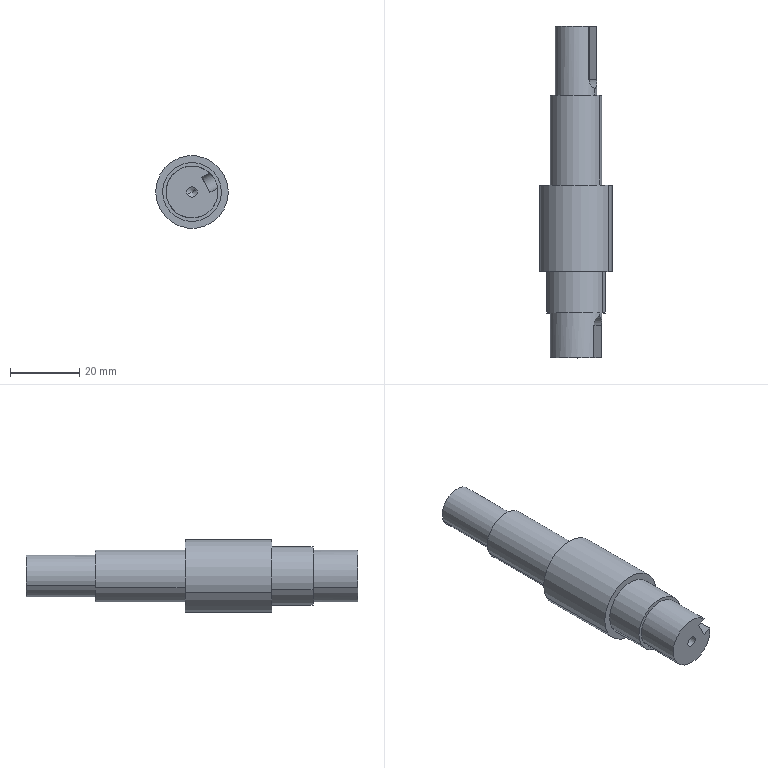Component | SolidWorks | GearIntermediateAxis-1 | 1 solid | 32 faces | box 21 x 96 x 21 mm | volume 19909 mm3 | cylinder 16 | plane 12 | cone 4 | commonest cylinder face diameters 3 x4 15 x4 17 x2 21 x2 12 x2 5 x2 | material 5154-O, Bar (SS)
build123d program:
from build123d import *

# Parameters (mm, degrees)
CUT_EXTRUDE1_DEPTH    = 3
CUT_EXTRUDE2_DEPTH    = 3
M3_TAPPED_HOLE1_D     = 3
M3_TAPPED_HOLE1_DEPTH = 15
M3_TAPPED_HOLE1_TIP   = 0.9013
M3_TAPPED_HOLE2_D     = 3
M3_TAPPED_HOLE2_DEPTH = 15
M3_TAPPED_HOLE2_TIP   = 0.9013


with BuildPart() as part:
    # Sketch1 → Revolve1 (revolve)
    with BuildSketch(Plane.XY, mode=Mode.PRIVATE) as revolve1_sk:
        Polygon((0, 96), (-6, 96), (-6, 76), (-7.5, 76), (-7.5, 50), (-10.5, 50), (-10.5, 25), (-8.5, 25), (-8.5, 13), (-7.5, 13), (-7.5, 0), (0, 0), align=None)
    revolve(revolve1_sk.sketch.rotate(Axis((0, 111.479, 0), (0, -1, 0)), 270), axis=Axis((0, 111.479, 0), (0, -1, 0)))

    # Sketch2 → Cut-Extrude1 (cut)
    with BuildSketch(Plane.XY.offset(6)):
        with BuildLine():
            Line((2.5, 96), (2.5, 80.5))
            ThreePointArc((2.5, 80.5), (0, 78), (-2.5, 80.5))
            Line((-2.5, 80.5), (-2.5, 96))
            ThreePointArc((-2.5, 96), (0, 98.5), (2.5, 96))
        make_face()
    extrude(amount=-CUT_EXTRUDE1_DEPTH, mode=Mode.SUBTRACT)

    # Sketch3 → Cut-Extrude2 (cut)
    with BuildSketch(Plane.XY.offset(7.5)):
        with BuildLine():
            Line((-2.5, 0), (-2.5, 9.5))
            ThreePointArc((-2.5, 9.5), (0, 12), (2.5, 9.5))
            Line((2.5, 9.5), (2.5, 0))
            ThreePointArc((2.5, 0), (0, -2.5), (-2.5, 0))
        make_face()
    extrude(amount=-CUT_EXTRUDE2_DEPTH, mode=Mode.SUBTRACT)

    # M3 Tapped Hole1
    with Locations(Plane(origin=(0, 96, 0), x_dir=(1, 0, 0), z_dir=(0, 1, 0))):
        with Locations((0, 0)):
            Hole(M3_TAPPED_HOLE1_D / 2, depth=M3_TAPPED_HOLE1_DEPTH)
            with Locations((0, 0, -(M3_TAPPED_HOLE1_DEPTH + M3_TAPPED_HOLE1_TIP / 2))):  # 118° drill point
                Cone(0, M3_TAPPED_HOLE1_D / 2, M3_TAPPED_HOLE1_TIP, mode=Mode.SUBTRACT)

    # M3 Tapped Hole2
    with Locations(Plane(origin=(0, 0, 0), x_dir=(-1, 0, 0), z_dir=(0, -1, 0))):
        with Locations((0, 0)):
            Hole(M3_TAPPED_HOLE2_D / 2, depth=M3_TAPPED_HOLE2_DEPTH)
            with Locations((0, 0, -(M3_TAPPED_HOLE2_DEPTH + M3_TAPPED_HOLE2_TIP / 2))):  # 118° drill point
                Cone(0, M3_TAPPED_HOLE2_D / 2, M3_TAPPED_HOLE2_TIP, mode=Mode.SUBTRACT)


solid = part.part

# Placed as in the assembly
solid = solid.moved(Location((-165.724, 61.266, -166.507), (0, 62.569, 0)))
STEP:
#1=COLOUR_RGB('',0.7922,0.8196,0.9333);
#2=FILL_AREA_STYLE_COLOUR('',#1);
#3=FILL_AREA_STYLE('',(#2));
#4=SURFACE_STYLE_FILL_AREA(#3);
#5=SURFACE_SIDE_STYLE('',(#4));
#6=SURFACE_STYLE_USAGE(.BOTH.,#5);
#7=PRESENTATION_STYLE_ASSIGNMENT((#6));
#8=CARTESIAN_POINT('',(-6.472,3.003,-6.528));
#9=VERTEX_POINT('',#8);
#10=CARTESIAN_POINT('',(-6.577,3.003,-6.583));
#11=VERTEX_POINT('',#10);
#12=CARTESIAN_POINT('',(-6.525,3.003,-6.555));
#13=DIRECTION('',(0.,-1.,0.));
#14=DIRECTION('',(-0.8876,0.,-0.4607));
#15=AXIS2_PLACEMENT_3D('',#12,#13,#14);
#16=CIRCLE('',#15,0.05906);
#17=EDGE_CURVE('',#9,#11,#16,.T.);
#18=ORIENTED_EDGE('',*,*,#17,.F.);
#19=CARTESIAN_POINT('',(-6.472,2.412,-6.528));
#20=VERTEX_POINT('',#19);
#21=CARTESIAN_POINT('',(-6.472,2.412,-6.528));
#22=DIRECTION('',(0.,-1.,0.));
#23=VECTOR('',#22,39.37);
#24=LINE('',#21,#23);
#25=EDGE_CURVE('',#9,#20,#24,.T.);
#26=ORIENTED_EDGE('',*,*,#25,.T.);
#27=CARTESIAN_POINT('',(-6.577,2.412,-6.583));
#28=VERTEX_POINT('',#27);
#29=CARTESIAN_POINT('',(-6.525,2.412,-6.555));
#30=DIRECTION('',(0.,-1.,0.));
#31=DIRECTION('',(-0.8876,0.,-0.4607));
#32=AXIS2_PLACEMENT_3D('',#29,#30,#31);
#33=CIRCLE('',#32,0.05906);
#34=EDGE_CURVE('',#20,#28,#33,.T.);
#35=ORIENTED_EDGE('',*,*,#34,.T.);
#36=CARTESIAN_POINT('',(-6.577,2.412,-6.583));
#37=DIRECTION('',(0.,-1.,0.));
#38=VECTOR('',#37,39.37);
#39=LINE('',#36,#38);
#40=EDGE_CURVE('',#11,#28,#39,.T.);
#41=ORIENTED_EDGE('',*,*,#40,.F.);
#42=EDGE_LOOP('',(#18,#26,#35,#41));
#43=FACE_OUTER_BOUND('',#42,.T.);
#44=CARTESIAN_POINT('',(-6.525,2.412,-6.555));
#45=DIRECTION('',(0.,-1.,0.));
#46=DIRECTION('',(-0.8876,0.,-0.4607));
#47=AXIS2_PLACEMENT_3D('',#44,#45,#46);
#48=CYLINDRICAL_SURFACE('',#47,0.05906);
#49=ADVANCED_FACE('',(#43),#48,.F.);
#50=CARTESIAN_POINT('',(-6.525,3.038,-6.555));
#51=VERTEX_POINT('',#50);
#52=CARTESIAN_POINT('',(-6.577,3.003,-6.583));
#53=DIRECTION('',(-0.7608,-0.515,-0.3949));
#54=VECTOR('',#53,39.37);
#55=LINE('',#52,#54);
#56=EDGE_CURVE('',#51,#11,#55,.T.);
#57=ORIENTED_EDGE('',*,*,#56,.F.);
#58=CARTESIAN_POINT('',(-6.472,3.003,-6.528));
#59=DIRECTION('',(0.7608,-0.515,0.3949));
#60=VECTOR('',#59,39.37);
#61=LINE('',#58,#60);
#62=EDGE_CURVE('',#51,#9,#61,.T.);
#63=ORIENTED_EDGE('',*,*,#62,.T.);
#64=ORIENTED_EDGE('',*,*,#17,.T.);
#65=EDGE_LOOP('',(#57,#63,#64));
#66=FACE_OUTER_BOUND('',#65,.T.);
#67=CARTESIAN_POINT('',(-6.525,3.003,-6.555));
#68=DIRECTION('',(0.,-1.,0.));
#69=DIRECTION('',(-0.8876,0.,-0.4607));
#70=AXIS2_PLACEMENT_3D('',#67,#68,#69);
#71=CONICAL_SURFACE('',#70,0.05906,1.03);
#72=ADVANCED_FACE('',(#66),#71,.F.);
#73=CARTESIAN_POINT('',(-6.577,5.601,-6.583));
#74=VERTEX_POINT('',#73);
#75=CARTESIAN_POINT('',(-6.472,5.601,-6.528));
#76=VERTEX_POINT('',#75);
#77=CARTESIAN_POINT('',(-6.525,5.601,-6.555));
#78=DIRECTION('',(0.,1.,0.));
#79=DIRECTION('',(0.8876,0.,0.4607));
#80=AXIS2_PLACEMENT_3D('',#77,#78,#79);
#81=CIRCLE('',#80,0.05906);
#82=EDGE_CURVE('',#74,#76,#81,.T.);
#83=ORIENTED_EDGE('',*,*,#82,.F.);
#84=CARTESIAN_POINT('',(-6.577,6.192,-6.583));
#85=VERTEX_POINT('',#84);
#86=CARTESIAN_POINT('',(-6.577,6.192,-6.583));
#87=DIRECTION('',(0.,1.,0.));
#88=VECTOR('',#87,39.37);
#89=LINE('',#86,#88);
#90=EDGE_CURVE('',#74,#85,#89,.T.);
#91=ORIENTED_EDGE('',*,*,#90,.T.);
#92=CARTESIAN_POINT('',(-6.472,6.192,-6.528));
#93=VERTEX_POINT('',#92);
#94=CARTESIAN_POINT('',(-6.525,6.192,-6.555));
#95=DIRECTION('',(0.,1.,0.));
#96=DIRECTION('',(0.8876,0.,0.4607));
#97=AXIS2_PLACEMENT_3D('',#94,#95,#96);
#98=CIRCLE('',#97,0.05906);
#99=EDGE_CURVE('',#85,#93,#98,.T.);
#100=ORIENTED_EDGE('',*,*,#99,.T.);
#101=CARTESIAN_POINT('',(-6.472,6.192,-6.528));
#102=DIRECTION('',(0.,1.,0.));
#103=VECTOR('',#102,39.37);
#104=LINE('',#101,#103);
#105=EDGE_CURVE('',#76,#93,#104,.T.);
#106=ORIENTED_EDGE('',*,*,#105,.F.);
#107=EDGE_LOOP('',(#83,#91,#100,#106));
#108=FACE_OUTER_BOUND('',#107,.T.);
#109=CARTESIAN_POINT('',(-6.525,6.192,-6.555));
#110=DIRECTION('',(0.,1.,0.));
#111=DIRECTION('',(0.8876,0.,0.4607));
#112=AXIS2_PLACEMENT_3D('',#109,#110,#111);
#113=CYLINDRICAL_SURFACE('',#112,0.05906);
#114=ADVANCED_FACE('',(#108),#113,.F.);
#115=CARTESIAN_POINT('',(-6.525,5.566,-6.555));
#116=VERTEX_POINT('',#115);
#117=CARTESIAN_POINT('',(-6.472,5.601,-6.528));
#118=DIRECTION('',(0.7608,0.515,0.3949));
#119=VECTOR('',#118,39.37);
#120=LINE('',#117,#119);
#121=EDGE_CURVE('',#116,#76,#120,.T.);
#122=ORIENTED_EDGE('',*,*,#121,.F.);
#123=CARTESIAN_POINT('',(-6.577,5.601,-6.583));
#124=DIRECTION('',(-0.7608,0.515,-0.3949));
#125=VECTOR('',#124,39.37);
#126=LINE('',#123,#125);
#127=EDGE_CURVE('',#116,#74,#126,.T.);
#128=ORIENTED_EDGE('',*,*,#127,.T.);
#129=ORIENTED_EDGE('',*,*,#82,.T.);
#130=EDGE_LOOP('',(#122,#128,#129));
#131=FACE_OUTER_BOUND('',#130,.T.);
#132=CARTESIAN_POINT('',(-6.525,5.601,-6.555));
#133=DIRECTION('',(0.,1.,0.));
#134=DIRECTION('',(0.8876,0.,0.4607));
#135=AXIS2_PLACEMENT_3D('',#132,#133,#134);
#136=CONICAL_SURFACE('',#135,0.05906,1.03);
#137=ADVANCED_FACE('',(#131),#136,.F.);
#138=CARTESIAN_POINT('',(-6.232,2.412,-6.515));
#139=VERTEX_POINT('',#138);
#140=CARTESIAN_POINT('',(-6.787,2.412,-6.691));
#141=VERTEX_POINT('',#140);
#142=CARTESIAN_POINT('',(-6.525,2.412,-6.555));
#143=DIRECTION('',(0.,1.,0.));
#144=DIRECTION('',(0.8876,0.,0.4607));
#145=AXIS2_PLACEMENT_3D('',#142,#143,#144);
#146=CIRCLE('',#145,0.2953);
#147=EDGE_CURVE('',#139,#141,#146,.T.);
#148=ORIENTED_EDGE('',*,*,#147,.T.);
#149=CARTESIAN_POINT('',(-6.787,2.924,-6.691));
#150=VERTEX_POINT('',#149);
#151=CARTESIAN_POINT('',(-6.787,6.801,-6.691));
#152=DIRECTION('',(0.,1.,0.));
#153=VECTOR('',#152,39.37);
#154=LINE('',#151,#153);
#155=EDGE_CURVE('',#141,#150,#154,.T.);
#156=ORIENTED_EDGE('',*,*,#155,.T.);
#157=CARTESIAN_POINT('',(-6.263,2.924,-6.419));
#158=VERTEX_POINT('',#157);
#159=CARTESIAN_POINT('',(-6.525,2.924,-6.555));
#160=DIRECTION('',(0.,1.,0.));
#161=DIRECTION('',(0.8876,0.,0.4607));
#162=AXIS2_PLACEMENT_3D('',#159,#160,#161);
#163=CIRCLE('',#162,0.2953);
#164=EDGE_CURVE('',#158,#150,#163,.T.);
#165=ORIENTED_EDGE('',*,*,#164,.F.);
#166=CARTESIAN_POINT('',(-6.263,2.884,-6.419));
#167=VERTEX_POINT('',#166);
#168=CARTESIAN_POINT('',(-6.263,6.801,-6.419));
#169=DIRECTION('',(0.,1.,0.));
#170=VECTOR('',#169,39.37);
#171=LINE('',#168,#170);
#172=EDGE_CURVE('',#167,#158,#171,.T.);
#173=ORIENTED_EDGE('',*,*,#172,.F.);
#174=CARTESIAN_POINT('',(-6.232,2.786,-6.515));
#175=VERTEX_POINT('',#174);
#176=CARTESIAN_POINT('',(-6.232,2.786,-6.515));
#177=CARTESIAN_POINT('',(-6.232,2.793,-6.515));
#178=CARTESIAN_POINT('',(-6.232,2.799,-6.514));
#179=CARTESIAN_POINT('',(-6.233,2.812,-6.511));
#180=CARTESIAN_POINT('',(-6.233,2.818,-6.509));
#181=CARTESIAN_POINT('',(-6.234,2.83,-6.504));
#182=CARTESIAN_POINT('',(-6.234,2.836,-6.501));
#183=CARTESIAN_POINT('',(-6.236,2.846,-6.494));
#184=CARTESIAN_POINT('',(-6.237,2.851,-6.489));
#185=CARTESIAN_POINT('',(-6.24,2.865,-6.476));
#186=CARTESIAN_POINT('',(-6.243,2.872,-6.465));
#187=CARTESIAN_POINT('',(-6.249,2.879,-6.448));
#188=CARTESIAN_POINT('',(-6.252,2.881,-6.443));
#189=CARTESIAN_POINT('',(-6.257,2.884,-6.431));
#190=CARTESIAN_POINT('',(-6.26,2.884,-6.425));
#191=CARTESIAN_POINT('',(-6.263,2.884,-6.419));
#192=B_SPLINE_CURVE_WITH_KNOTS('',3,(#176,#177,#178,#179,#180,#181,#182,#183,#184,#185,#186,#187,#188,#189,#190,#191),.UNSPECIFIED.,.F.,.F.,(4,2,2,2,2,2,2,4),(0.,0.0004922,0.0009844,0.001477,0.001969,0.002953,0.003445,0.003937),.UNSPECIFIED.);
#193=EDGE_CURVE('',#175,#167,#192,.T.);
#194=ORIENTED_EDGE('',*,*,#193,.F.);
#195=CARTESIAN_POINT('',(-6.232,6.801,-6.515));
#196=DIRECTION('',(0.,1.,0.));
#197=VECTOR('',#196,39.37);
#198=LINE('',#195,#197);
#199=EDGE_CURVE('',#139,#175,#198,.T.);
#200=ORIENTED_EDGE('',*,*,#199,.F.);
#201=EDGE_LOOP('',(#148,#156,#165,#173,#194,#200));
#202=FACE_OUTER_BOUND('',#201,.T.);
#203=CARTESIAN_POINT('',(-6.525,6.801,-6.555));
#204=DIRECTION('',(0.,1.,0.));
#205=DIRECTION('',(0.8876,0.,0.4607));
#206=AXIS2_PLACEMENT_3D('',#203,#204,#205);
#207=CYLINDRICAL_SURFACE('',#206,0.2953);
#208=ADVANCED_FACE('',(#202),#207,.T.);
#209=CARTESIAN_POINT('',(-6.228,2.924,-6.401));
#210=VERTEX_POINT('',#209);
#211=CARTESIAN_POINT('',(-6.822,2.924,-6.71));
#212=VERTEX_POINT('',#211);
#213=CARTESIAN_POINT('',(-6.525,2.924,-6.555));
#214=DIRECTION('',(0.,1.,0.));
#215=DIRECTION('',(0.8876,0.,0.4607));
#216=AXIS2_PLACEMENT_3D('',#213,#214,#215);
#217=CIRCLE('',#216,0.3346);
#218=EDGE_CURVE('',#210,#212,#217,.T.);
#219=ORIENTED_EDGE('',*,*,#218,.T.);
#220=CARTESIAN_POINT('',(-6.822,3.396,-6.71));
#221=VERTEX_POINT('',#220);
#222=CARTESIAN_POINT('',(-6.822,6.801,-6.71));
#223=DIRECTION('',(0.,1.,0.));
#224=VECTOR('',#223,39.37);
#225=LINE('',#222,#224);
#226=EDGE_CURVE('',#212,#221,#225,.T.);
#227=ORIENTED_EDGE('',*,*,#226,.T.);
#228=CARTESIAN_POINT('',(-6.228,3.396,-6.401));
#229=VERTEX_POINT('',#228);
#230=CARTESIAN_POINT('',(-6.525,3.396,-6.555));
#231=DIRECTION('',(0.,1.,0.));
#232=DIRECTION('',(0.8876,0.,0.4607));
#233=AXIS2_PLACEMENT_3D('',#230,#231,#232);
#234=CIRCLE('',#233,0.3346);
#235=EDGE_CURVE('',#229,#221,#234,.T.);
#236=ORIENTED_EDGE('',*,*,#235,.F.);
#237=CARTESIAN_POINT('',(-6.228,6.801,-6.401));
#238=DIRECTION('',(0.,1.,0.));
#239=VECTOR('',#238,39.37);
#240=LINE('',#237,#239);
#241=EDGE_CURVE('',#210,#229,#240,.T.);
#242=ORIENTED_EDGE('',*,*,#241,.F.);
#243=EDGE_LOOP('',(#219,#227,#236,#242));
#244=FACE_OUTER_BOUND('',#243,.T.);
#245=CARTESIAN_POINT('',(-6.525,6.801,-6.555));
#246=DIRECTION('',(0.,1.,0.));
#247=DIRECTION('',(0.8876,0.,0.4607));
#248=AXIS2_PLACEMENT_3D('',#245,#246,#247);
#249=CYLINDRICAL_SURFACE('',#248,0.3346);
#250=ADVANCED_FACE('',(#244),#249,.T.);
#251=CARTESIAN_POINT('',(-6.158,3.396,-6.365));
#252=VERTEX_POINT('',#251);
#253=CARTESIAN_POINT('',(-6.891,3.396,-6.746));
#254=VERTEX_POINT('',#253);
#255=CARTESIAN_POINT('',(-6.525,3.396,-6.555));
#256=DIRECTION('',(0.,1.,0.));
#257=DIRECTION('',(0.8876,0.,0.4607));
#258=AXIS2_PLACEMENT_3D('',#255,#256,#257);
#259=CIRCLE('',#258,0.4134);
#260=EDGE_CURVE('',#252,#254,#259,.T.);
#261=ORIENTED_EDGE('',*,*,#260,.T.);
#262=CARTESIAN_POINT('',(-6.891,4.381,-6.746));
#263=VERTEX_POINT('',#262);
#264=CARTESIAN_POINT('',(-6.891,6.801,-6.746));
#265=DIRECTION('',(0.,1.,0.));
#266=VECTOR('',#265,39.37);
#267=LINE('',#264,#266);
#268=EDGE_CURVE('',#254,#263,#267,.T.);
#269=ORIENTED_EDGE('',*,*,#268,.T.);
#270=CARTESIAN_POINT('',(-6.158,4.381,-6.365));
#271=VERTEX_POINT('',#270);
#272=CARTESIAN_POINT('',(-6.525,4.381,-6.555));
#273=DIRECTION('',(0.,1.,0.));
#274=DIRECTION('',(0.8876,0.,0.4607));
#275=AXIS2_PLACEMENT_3D('',#272,#273,#274);
#276=CIRCLE('',#275,0.4134);
#277=EDGE_CURVE('',#271,#263,#276,.T.);
#278=ORIENTED_EDGE('',*,*,#277,.F.);
#279=CARTESIAN_POINT('',(-6.158,6.801,-6.365));
#280=DIRECTION('',(0.,1.,0.));
#281=VECTOR('',#280,39.37);
#282=LINE('',#279,#281);
#283=EDGE_CURVE('',#252,#271,#282,.T.);
#284=ORIENTED_EDGE('',*,*,#283,.F.);
#285=EDGE_LOOP('',(#261,#269,#278,#284));
#286=FACE_OUTER_BOUND('',#285,.T.);
#287=CARTESIAN_POINT('',(-6.525,6.801,-6.555));
#288=DIRECTION('',(0.,1.,0.));
#289=DIRECTION('',(0.8876,0.,0.4607));
#290=AXIS2_PLACEMENT_3D('',#287,#288,#289);
#291=CYLINDRICAL_SURFACE('',#290,0.4134);
#292=ADVANCED_FACE('',(#286),#291,.T.);
#293=CARTESIAN_POINT('',(-6.263,4.381,-6.419));
#294=VERTEX_POINT('',#293);
#295=CARTESIAN_POINT('',(-6.787,4.381,-6.691));
#296=VERTEX_POINT('',#295);
#297=CARTESIAN_POINT('',(-6.525,4.381,-6.555));
#298=DIRECTION('',(0.,1.,0.));
#299=DIRECTION('',(0.8876,0.,0.4607));
#300=AXIS2_PLACEMENT_3D('',#297,#298,#299);
#301=CIRCLE('',#300,0.2953);
#302=EDGE_CURVE('',#294,#296,#301,.T.);
#303=ORIENTED_EDGE('',*,*,#302,.T.);
#304=CARTESIAN_POINT('',(-6.787,5.404,-6.691));
#305=VERTEX_POINT('',#304);
#306=CARTESIAN_POINT('',(-6.787,6.801,-6.691));
#307=DIRECTION('',(0.,1.,0.));
#308=VECTOR('',#307,39.37);
#309=LINE('',#306,#308);
#310=EDGE_CURVE('',#296,#305,#309,.T.);
#311=ORIENTED_EDGE('',*,*,#310,.T.);
#312=CARTESIAN_POINT('',(-6.263,5.404,-6.419));
#313=VERTEX_POINT('',#312);
#314=CARTESIAN_POINT('',(-6.525,5.404,-6.555));
#315=DIRECTION('',(0.,1.,0.));
#316=DIRECTION('',(0.8876,0.,0.4607));
#317=AXIS2_PLACEMENT_3D('',#314,#315,#316);
#318=CIRCLE('',#317,0.2953);
#319=EDGE_CURVE('',#313,#305,#318,.T.);
#320=ORIENTED_EDGE('',*,*,#319,.F.);
#321=CARTESIAN_POINT('',(-6.263,6.801,-6.419));
#322=DIRECTION('',(0.,1.,0.));
#323=VECTOR('',#322,39.37);
#324=LINE('',#321,#323);
#325=EDGE_CURVE('',#294,#313,#324,.T.);
#326=ORIENTED_EDGE('',*,*,#325,.F.);
#327=EDGE_LOOP('',(#303,#311,#320,#326));
#328=FACE_OUTER_BOUND('',#327,.T.);
#329=CARTESIAN_POINT('',(-6.525,6.801,-6.555));
#330=DIRECTION('',(0.,1.,0.));
#331=DIRECTION('',(0.8876,0.,0.4607));
#332=AXIS2_PLACEMENT_3D('',#329,#330,#331);
#333=CYLINDRICAL_SURFACE('',#332,0.2953);
#334=ADVANCED_FACE('',(#328),#333,.T.);
#335=CARTESIAN_POINT('',(-6.315,5.404,-6.447));
#336=VERTEX_POINT('',#335);
#337=CARTESIAN_POINT('',(-6.734,5.404,-6.664));
#338=VERTEX_POINT('',#337);
#339=CARTESIAN_POINT('',(-6.525,5.404,-6.555));
#340=DIRECTION('',(0.,1.,0.));
#341=DIRECTION('',(0.8876,0.,0.4607));
#342=AXIS2_PLACEMENT_3D('',#339,#340,#341);
#343=CIRCLE('',#342,0.2362);
#344=EDGE_CURVE('',#336,#338,#343,.T.);
#345=ORIENTED_EDGE('',*,*,#344,.T.);
#346=CARTESIAN_POINT('',(-6.734,6.192,-6.664));
#347=VERTEX_POINT('',#346);
#348=CARTESIAN_POINT('',(-6.734,6.801,-6.664));
#349=DIRECTION('',(0.,1.,0.));
#350=VECTOR('',#349,39.37);
#351=LINE('',#348,#350);
#352=EDGE_CURVE('',#338,#347,#351,.T.);
#353=ORIENTED_EDGE('',*,*,#352,.T.);
#354=CARTESIAN_POINT('',(-6.289,6.192,-6.544));
#355=VERTEX_POINT('',#354);
#356=CARTESIAN_POINT('',(-6.525,6.192,-6.555));
#357=DIRECTION('',(0.,1.,0.));
#358=DIRECTION('',(0.8876,0.,0.4607));
#359=AXIS2_PLACEMENT_3D('',#356,#357,#358);
#360=CIRCLE('',#359,0.2362);
#361=EDGE_CURVE('',#355,#347,#360,.T.);
#362=ORIENTED_EDGE('',*,*,#361,.F.);
#363=CARTESIAN_POINT('',(-6.289,5.581,-6.544));
#364=VERTEX_POINT('',#363);
#365=CARTESIAN_POINT('',(-6.289,6.801,-6.544));
#366=DIRECTION('',(0.,1.,0.));
#367=VECTOR('',#366,39.37);
#368=LINE('',#365,#367);
#369=EDGE_CURVE('',#364,#355,#368,.T.);
#370=ORIENTED_EDGE('',*,*,#369,.F.);
#371=CARTESIAN_POINT('',(-6.315,5.483,-6.447));
#372=VERTEX_POINT('',#371);
#373=CARTESIAN_POINT('',(-6.315,5.483,-6.447));
#374=CARTESIAN_POINT('',(-6.312,5.483,-6.452));
#375=CARTESIAN_POINT('',(-6.309,5.484,-6.458));
#376=CARTESIAN_POINT('',(-6.304,5.486,-6.47));
#377=CARTESIAN_POINT('',(-6.302,5.488,-6.476));
#378=CARTESIAN_POINT('',(-6.298,5.493,-6.487));
#379=CARTESIAN_POINT('',(-6.297,5.496,-6.493));
#380=CARTESIAN_POINT('',(-6.294,5.503,-6.504));
#381=CARTESIAN_POINT('',(-6.293,5.507,-6.509));
#382=CARTESIAN_POINT('',(-6.291,5.516,-6.518));
#383=CARTESIAN_POINT('',(-6.291,5.521,-6.522));
#384=CARTESIAN_POINT('',(-6.29,5.532,-6.53));
#385=CARTESIAN_POINT('',(-6.289,5.537,-6.533));
#386=CARTESIAN_POINT('',(-6.289,5.555,-6.541));
#387=CARTESIAN_POINT('',(-6.289,5.568,-6.544));
#388=CARTESIAN_POINT('',(-6.289,5.581,-6.544));
#389=B_SPLINE_CURVE_WITH_KNOTS('',3,(#373,#374,#375,#376,#377,#378,#379,#380,#381,#382,#383,#384,#385,#386,#387,#388),.UNSPECIFIED.,.F.,.F.,(4,2,2,2,2,2,2,4),(0.003955,0.004448,0.004942,0.005435,0.005929,0.006423,0.006916,0.007903),.UNSPECIFIED.);
#390=EDGE_CURVE('',#372,#364,#389,.T.);
#391=ORIENTED_EDGE('',*,*,#390,.F.);
#392=CARTESIAN_POINT('',(-6.315,6.801,-6.447));
#393=DIRECTION('',(0.,1.,0.));
#394=VECTOR('',#393,39.37);
#395=LINE('',#392,#394);
#396=EDGE_CURVE('',#336,#372,#395,.T.);
#397=ORIENTED_EDGE('',*,*,#396,.F.);
#398=EDGE_LOOP('',(#345,#353,#362,#370,#391,#397));
#399=FACE_OUTER_BOUND('',#398,.T.);
#400=CARTESIAN_POINT('',(-6.525,6.801,-6.555));
#401=DIRECTION('',(0.,1.,0.));
#402=DIRECTION('',(0.8876,0.,0.4607));
#403=AXIS2_PLACEMENT_3D('',#400,#401,#402);
#404=CYLINDRICAL_SURFACE('',#403,0.2362);
#405=ADVANCED_FACE('',(#399),#404,.T.);
#406=CARTESIAN_POINT('',(-6.525,6.192,-6.555));
#407=DIRECTION('',(0.,1.,0.));
#408=DIRECTION('',(0.8876,0.,0.4607));
#409=AXIS2_PLACEMENT_3D('',#406,#407,#408);
#410=CIRCLE('',#409,0.05906);
#411=EDGE_CURVE('',#93,#85,#410,.T.);
#412=ORIENTED_EDGE('',*,*,#411,.F.);
#413=ORIENTED_EDGE('',*,*,#99,.F.);
#414=EDGE_LOOP('',(#412,#413));
#415=FACE_BOUND('',#414,.T.);
#416=CARTESIAN_POINT('',(-6.374,6.192,-6.588));
#417=VERTEX_POINT('',#416);
#418=CARTESIAN_POINT('',(-6.374,6.192,-6.588));
#419=DIRECTION('',(0.8876,0.,0.4607));
#420=VECTOR('',#419,39.37);
#421=LINE('',#418,#420);
#422=EDGE_CURVE('',#417,#355,#421,.T.);
#423=ORIENTED_EDGE('',*,*,#422,.T.);
#424=ORIENTED_EDGE('',*,*,#361,.T.);
#425=CARTESIAN_POINT('',(-6.379,6.192,-6.369));
#426=VERTEX_POINT('',#425);
#427=CARTESIAN_POINT('',(-6.525,6.192,-6.555));
#428=DIRECTION('',(0.,1.,0.));
#429=DIRECTION('',(0.8876,0.,0.4607));
#430=AXIS2_PLACEMENT_3D('',#427,#428,#429);
#431=CIRCLE('',#430,0.2362);
#432=EDGE_CURVE('',#347,#426,#431,.T.);
#433=ORIENTED_EDGE('',*,*,#432,.T.);
#434=CARTESIAN_POINT('',(-6.465,6.192,-6.414));
#435=VERTEX_POINT('',#434);
#436=CARTESIAN_POINT('',(-6.465,6.192,-6.414));
#437=DIRECTION('',(0.8876,0.,0.4607));
#438=VECTOR('',#437,39.37);
#439=LINE('',#436,#438);
#440=EDGE_CURVE('',#435,#426,#439,.T.);
#441=ORIENTED_EDGE('',*,*,#440,.F.);
#442=CARTESIAN_POINT('',(-6.42,6.192,-6.501));
#443=DIRECTION('',(0.4607,0.,-0.8876));
#444=VECTOR('',#443,39.37);
#445=LINE('',#442,#444);
#446=EDGE_CURVE('',#435,#417,#445,.T.);
#447=ORIENTED_EDGE('',*,*,#446,.T.);
#448=EDGE_LOOP('',(#423,#424,#433,#441,#447));
#449=FACE_OUTER_BOUND('',#448,.T.);
#450=CARTESIAN_POINT('',(-6.525,6.192,-6.555));
#451=DIRECTION('',(0.,1.,0.));
#452=DIRECTION('',(0.8876,0.,0.4607));
#453=AXIS2_PLACEMENT_3D('',#450,#451,#452);
#454=PLANE('',#453);
#455=ADVANCED_FACE('',(#415,#449),#454,.T.);
#456=ORIENTED_EDGE('',*,*,#352,.F.);
#457=CARTESIAN_POINT('',(-6.525,5.404,-6.555));
#458=DIRECTION('',(0.,1.,0.));
#459=DIRECTION('',(0.8876,0.,0.4607));
#460=AXIS2_PLACEMENT_3D('',#457,#458,#459);
#461=CIRCLE('',#460,0.2362);
#462=EDGE_CURVE('',#338,#336,#461,.T.);
#463=ORIENTED_EDGE('',*,*,#462,.T.);
#464=ORIENTED_EDGE('',*,*,#396,.T.);
#465=CARTESIAN_POINT('',(-6.379,5.581,-6.369));
#466=VERTEX_POINT('',#465);
#467=CARTESIAN_POINT('',(-6.379,5.581,-6.369));
#468=CARTESIAN_POINT('',(-6.379,5.575,-6.369));
#469=CARTESIAN_POINT('',(-6.379,5.568,-6.37));
#470=CARTESIAN_POINT('',(-6.377,5.556,-6.371));
#471=CARTESIAN_POINT('',(-6.375,5.549,-6.373));
#472=CARTESIAN_POINT('',(-6.371,5.537,-6.376));
#473=CARTESIAN_POINT('',(-6.368,5.532,-6.378));
#474=CARTESIAN_POINT('',(-6.363,5.521,-6.383));
#475=CARTESIAN_POINT('',(-6.36,5.516,-6.386));
#476=CARTESIAN_POINT('',(-6.35,5.503,-6.396));
#477=CARTESIAN_POINT('',(-6.342,5.495,-6.405));
#478=CARTESIAN_POINT('',(-6.332,5.488,-6.419));
#479=CARTESIAN_POINT('',(-6.328,5.486,-6.424));
#480=CARTESIAN_POINT('',(-6.321,5.484,-6.435));
#481=CARTESIAN_POINT('',(-6.318,5.483,-6.441));
#482=CARTESIAN_POINT('',(-6.315,5.483,-6.447));
#483=B_SPLINE_CURVE_WITH_KNOTS('',3,(#467,#468,#469,#470,#471,#472,#473,#474,#475,#476,#477,#478,#479,#480,#481,#482),.UNSPECIFIED.,.F.,.F.,(4,2,2,2,2,2,2,4),(0.,0.0004943,0.0009887,0.001483,0.001977,0.002966,0.00346,0.003955),.UNSPECIFIED.);
#484=EDGE_CURVE('',#466,#372,#483,.T.);
#485=ORIENTED_EDGE('',*,*,#484,.F.);
#486=CARTESIAN_POINT('',(-6.379,6.801,-6.369));
#487=DIRECTION('',(0.,-1.,0.));
#488=VECTOR('',#487,39.37);
#489=LINE('',#486,#488);
#490=EDGE_CURVE('',#426,#466,#489,.T.);
#491=ORIENTED_EDGE('',*,*,#490,.F.);
#492=ORIENTED_EDGE('',*,*,#432,.F.);
#493=EDGE_LOOP('',(#456,#463,#464,#485,#491,#492));
#494=FACE_OUTER_BOUND('',#493,.T.);
#495=CARTESIAN_POINT('',(-6.525,6.801,-6.555));
#496=DIRECTION('',(0.,1.,0.));
#497=DIRECTION('',(0.8876,0.,0.4607));
#498=AXIS2_PLACEMENT_3D('',#495,#496,#497);
#499=CYLINDRICAL_SURFACE('',#498,0.2362);
#500=ADVANCED_FACE('',(#494),#499,.T.);
#501=ORIENTED_EDGE('',*,*,#319,.T.);
#502=CARTESIAN_POINT('',(-6.525,5.404,-6.555));
#503=DIRECTION('',(0.,1.,0.));
#504=DIRECTION('',(0.8876,0.,0.4607));
#505=AXIS2_PLACEMENT_3D('',#502,#503,#504);
#506=CIRCLE('',#505,0.2953);
#507=EDGE_CURVE('',#305,#313,#506,.T.);
#508=ORIENTED_EDGE('',*,*,#507,.T.);
#509=EDGE_LOOP('',(#501,#508));
#510=FACE_OUTER_BOUND('',#509,.T.);
#511=ORIENTED_EDGE('',*,*,#344,.F.);
#512=ORIENTED_EDGE('',*,*,#462,.F.);
#513=EDGE_LOOP('',(#511,#512));
#514=FACE_BOUND('',#513,.T.);
#515=CARTESIAN_POINT('',(-6.633,5.404,-6.346));
#516=DIRECTION('',(0.,1.,0.));
#517=DIRECTION('',(0.8876,0.,0.4607));
#518=AXIS2_PLACEMENT_3D('',#515,#516,#517);
#519=PLANE('',#518);
#520=ADVANCED_FACE('',(#510,#514),#519,.T.);
#521=ORIENTED_EDGE('',*,*,#310,.F.);
#522=CARTESIAN_POINT('',(-6.525,4.381,-6.555));
#523=DIRECTION('',(0.,1.,0.));
#524=DIRECTION('',(0.8876,0.,0.4607));
#525=AXIS2_PLACEMENT_3D('',#522,#523,#524);
#526=CIRCLE('',#525,0.2953);
#527=EDGE_CURVE('',#296,#294,#526,.T.);
#528=ORIENTED_EDGE('',*,*,#527,.T.);
#529=ORIENTED_EDGE('',*,*,#325,.T.);
#530=ORIENTED_EDGE('',*,*,#507,.F.);
#531=EDGE_LOOP('',(#521,#528,#529,#530));
#532=FACE_OUTER_BOUND('',#531,.T.);
#533=CARTESIAN_POINT('',(-6.525,6.801,-6.555));
#534=DIRECTION('',(0.,1.,0.));
#535=DIRECTION('',(0.8876,0.,0.4607));
#536=AXIS2_PLACEMENT_3D('',#533,#534,#535);
#537=CYLINDRICAL_SURFACE('',#536,0.2953);
#538=ADVANCED_FACE('',(#532),#537,.T.);
#539=ORIENTED_EDGE('',*,*,#277,.T.);
#540=CARTESIAN_POINT('',(-6.525,4.381,-6.555));
#541=DIRECTION('',(0.,1.,0.));
#542=DIRECTION('',(0.8876,0.,0.4607));
#543=AXIS2_PLACEMENT_3D('',#540,#541,#542);
#544=CIRCLE('',#543,0.4134);
#545=EDGE_CURVE('',#263,#271,#544,.T.);
#546=ORIENTED_EDGE('',*,*,#545,.T.);
#547=EDGE_LOOP('',(#539,#546));
#548=FACE_OUTER_BOUND('',#547,.T.);
#549=ORIENTED_EDGE('',*,*,#302,.F.);
#550=ORIENTED_EDGE('',*,*,#527,.F.);
#551=EDGE_LOOP('',(#549,#550));
#552=FACE_BOUND('',#551,.T.);
#553=CARTESIAN_POINT('',(-6.661,4.381,-6.293));
#554=DIRECTION('',(0.,1.,0.));
#555=DIRECTION('',(0.8876,0.,0.4607));
#556=AXIS2_PLACEMENT_3D('',#553,#554,#555);
#557=PLANE('',#556);
#558=ADVANCED_FACE('',(#548,#552),#557,.T.);
#559=ORIENTED_EDGE('',*,*,#268,.F.);
#560=CARTESIAN_POINT('',(-6.525,3.396,-6.555));
#561=DIRECTION('',(0.,1.,0.));
#562=DIRECTION('',(0.8876,0.,0.4607));
#563=AXIS2_PLACEMENT_3D('',#560,#561,#562);
#564=CIRCLE('',#563,0.4134);
#565=EDGE_CURVE('',#254,#252,#564,.T.);
#566=ORIENTED_EDGE('',*,*,#565,.T.);
#567=ORIENTED_EDGE('',*,*,#283,.T.);
#568=ORIENTED_EDGE('',*,*,#545,.F.);
#569=EDGE_LOOP('',(#559,#566,#567,#568));
#570=FACE_OUTER_BOUND('',#569,.T.);
#571=CARTESIAN_POINT('',(-6.525,6.801,-6.555));
#572=DIRECTION('',(0.,1.,0.));
#573=DIRECTION('',(0.8876,0.,0.4607));
#574=AXIS2_PLACEMENT_3D('',#571,#572,#573);
#575=CYLINDRICAL_SURFACE('',#574,0.4134);
#576=ADVANCED_FACE('',(#570),#575,.T.);
#577=ORIENTED_EDGE('',*,*,#235,.T.);
#578=CARTESIAN_POINT('',(-6.525,3.396,-6.555));
#579=DIRECTION('',(0.,1.,0.));
#580=DIRECTION('',(0.8876,0.,0.4607));
#581=AXIS2_PLACEMENT_3D('',#578,#579,#580);
#582=CIRCLE('',#581,0.3346);
#583=EDGE_CURVE('',#221,#229,#582,.T.);
#584=ORIENTED_EDGE('',*,*,#583,.T.);
#585=EDGE_LOOP('',(#577,#584));
#586=FACE_BOUND('',#585,.T.);
#587=ORIENTED_EDGE('',*,*,#260,.F.);
#588=ORIENTED_EDGE('',*,*,#565,.F.);
#589=EDGE_LOOP('',(#587,#588));
#590=FACE_OUTER_BOUND('',#589,.T.);
#591=CARTESIAN_POINT('',(-6.715,3.396,-6.188));
#592=DIRECTION('',(0.,-1.,0.));
#593=DIRECTION('',(-0.8876,0.,-0.4607));
#594=AXIS2_PLACEMENT_3D('',#591,#592,#593);
#595=PLANE('',#594);
#596=ADVANCED_FACE('',(#586,#590),#595,.T.);
#597=ORIENTED_EDGE('',*,*,#226,.F.);
#598=CARTESIAN_POINT('',(-6.525,2.924,-6.555));
#599=DIRECTION('',(0.,1.,0.));
#600=DIRECTION('',(0.8876,0.,0.4607));
#601=AXIS2_PLACEMENT_3D('',#598,#599,#600);
#602=CIRCLE('',#601,0.3346);
#603=EDGE_CURVE('',#212,#210,#602,.T.);
#604=ORIENTED_EDGE('',*,*,#603,.T.);
#605=ORIENTED_EDGE('',*,*,#241,.T.);
#606=ORIENTED_EDGE('',*,*,#583,.F.);
#607=EDGE_LOOP('',(#597,#604,#605,#606));
#608=FACE_OUTER_BOUND('',#607,.T.);
#609=CARTESIAN_POINT('',(-6.525,6.801,-6.555));
#610=DIRECTION('',(0.,1.,0.));
#611=DIRECTION('',(0.8876,0.,0.4607));
#612=AXIS2_PLACEMENT_3D('',#609,#610,#611);
#613=CYLINDRICAL_SURFACE('',#612,0.3346);
#614=ADVANCED_FACE('',(#608),#613,.T.);
#615=ORIENTED_EDGE('',*,*,#164,.T.);
#616=CARTESIAN_POINT('',(-6.525,2.924,-6.555));
#617=DIRECTION('',(0.,1.,0.));
#618=DIRECTION('',(0.8876,0.,0.4607));
#619=AXIS2_PLACEMENT_3D('',#616,#617,#618);
#620=CIRCLE('',#619,0.2953);
#621=EDGE_CURVE('',#150,#158,#620,.T.);
#622=ORIENTED_EDGE('',*,*,#621,.T.);
#623=EDGE_LOOP('',(#615,#622));
#624=FACE_BOUND('',#623,.T.);
#625=ORIENTED_EDGE('',*,*,#218,.F.);
#626=ORIENTED_EDGE('',*,*,#603,.F.);
#627=EDGE_LOOP('',(#625,#626));
#628=FACE_OUTER_BOUND('',#627,.T.);
#629=CARTESIAN_POINT('',(-6.679,2.924,-6.258));
#630=DIRECTION('',(0.,-1.,0.));
#631=DIRECTION('',(-0.8876,0.,-0.4607));
#632=AXIS2_PLACEMENT_3D('',#629,#630,#631);
#633=PLANE('',#632);
#634=ADVANCED_FACE('',(#624,#628),#633,.T.);
#635=ORIENTED_EDGE('',*,*,#155,.F.);
#636=CARTESIAN_POINT('',(-6.323,2.412,-6.34));
#637=VERTEX_POINT('',#636);
#638=CARTESIAN_POINT('',(-6.525,2.412,-6.555));
#639=DIRECTION('',(0.,1.,0.));
#640=DIRECTION('',(0.8876,0.,0.4607));
#641=AXIS2_PLACEMENT_3D('',#638,#639,#640);
#642=CIRCLE('',#641,0.2953);
#643=EDGE_CURVE('',#141,#637,#642,.T.);
#644=ORIENTED_EDGE('',*,*,#643,.T.);
#645=CARTESIAN_POINT('',(-6.323,2.786,-6.34));
#646=VERTEX_POINT('',#645);
#647=CARTESIAN_POINT('',(-6.323,6.801,-6.34));
#648=DIRECTION('',(0.,-1.,0.));
#649=VECTOR('',#648,39.37);
#650=LINE('',#647,#649);
#651=EDGE_CURVE('',#646,#637,#650,.T.);
#652=ORIENTED_EDGE('',*,*,#651,.F.);
#653=CARTESIAN_POINT('',(-6.263,2.884,-6.419));
#654=CARTESIAN_POINT('',(-6.265,2.884,-6.414));
#655=CARTESIAN_POINT('',(-6.269,2.884,-6.408));
#656=CARTESIAN_POINT('',(-6.275,2.881,-6.397));
#657=CARTESIAN_POINT('',(-6.279,2.879,-6.392));
#658=CARTESIAN_POINT('',(-6.286,2.874,-6.382));
#659=CARTESIAN_POINT('',(-6.289,2.871,-6.377));
#660=CARTESIAN_POINT('',(-6.296,2.864,-6.369));
#661=CARTESIAN_POINT('',(-6.299,2.86,-6.365));
#662=CARTESIAN_POINT('',(-6.305,2.851,-6.358));
#663=CARTESIAN_POINT('',(-6.308,2.846,-6.355));
#664=CARTESIAN_POINT('',(-6.313,2.836,-6.349));
#665=CARTESIAN_POINT('',(-6.315,2.83,-6.347));
#666=CARTESIAN_POINT('',(-6.319,2.818,-6.344));
#667=CARTESIAN_POINT('',(-6.32,2.812,-6.342));
#668=CARTESIAN_POINT('',(-6.322,2.799,-6.34));
#669=CARTESIAN_POINT('',(-6.323,2.793,-6.34));
#670=CARTESIAN_POINT('',(-6.323,2.786,-6.34));
#671=B_SPLINE_CURVE_WITH_KNOTS('',3,(#653,#654,#655,#656,#657,#658,#659,#660,#661,#662,#663,#664,#665,#666,#667,#668,#669,#670),.UNSPECIFIED.,.F.,.F.,(4,2,2,2,2,2,2,2,4),(0.003937,0.004429,0.004921,0.005412,0.005904,0.006395,0.006887,0.007378,0.00787),.UNSPECIFIED.);
#672=EDGE_CURVE('',#167,#646,#671,.T.);
#673=ORIENTED_EDGE('',*,*,#672,.F.);
#674=ORIENTED_EDGE('',*,*,#172,.T.);
#675=ORIENTED_EDGE('',*,*,#621,.F.);
#676=EDGE_LOOP('',(#635,#644,#652,#673,#674,#675));
#677=FACE_OUTER_BOUND('',#676,.T.);
#678=CARTESIAN_POINT('',(-6.525,6.801,-6.555));
#679=DIRECTION('',(0.,1.,0.));
#680=DIRECTION('',(0.8876,0.,0.4607));
#681=AXIS2_PLACEMENT_3D('',#678,#679,#680);
#682=CYLINDRICAL_SURFACE('',#681,0.2953);
#683=ADVANCED_FACE('',(#677),#682,.T.);
#684=CARTESIAN_POINT('',(-6.525,2.412,-6.555));
#685=DIRECTION('',(0.,-1.,0.));
#686=DIRECTION('',(-0.8876,0.,-0.4607));
#687=AXIS2_PLACEMENT_3D('',#684,#685,#686);
#688=CIRCLE('',#687,0.05906);
#689=EDGE_CURVE('',#28,#20,#688,.T.);
#690=ORIENTED_EDGE('',*,*,#689,.F.);
#691=ORIENTED_EDGE('',*,*,#34,.F.);
#692=EDGE_LOOP('',(#690,#691));
#693=FACE_BOUND('',#692,.T.);
#694=CARTESIAN_POINT('',(-6.413,2.412,-6.386));
#695=VERTEX_POINT('',#694);
#696=CARTESIAN_POINT('',(-6.413,2.412,-6.386));
#697=DIRECTION('',(0.8876,0.,0.4607));
#698=VECTOR('',#697,39.37);
#699=LINE('',#696,#698);
#700=EDGE_CURVE('',#695,#637,#699,.T.);
#701=ORIENTED_EDGE('',*,*,#700,.T.);
#702=ORIENTED_EDGE('',*,*,#643,.F.);
#703=ORIENTED_EDGE('',*,*,#147,.F.);
#704=CARTESIAN_POINT('',(-6.322,2.412,-6.561));
#705=VERTEX_POINT('',#704);
#706=CARTESIAN_POINT('',(-6.322,2.412,-6.561));
#707=DIRECTION('',(0.8876,0.,0.4607));
#708=VECTOR('',#707,39.37);
#709=LINE('',#706,#708);
#710=EDGE_CURVE('',#705,#139,#709,.T.);
#711=ORIENTED_EDGE('',*,*,#710,.F.);
#712=CARTESIAN_POINT('',(-6.503,2.412,-6.212));
#713=DIRECTION('',(-0.4607,0.,0.8876));
#714=VECTOR('',#713,39.37);
#715=LINE('',#712,#714);
#716=EDGE_CURVE('',#705,#695,#715,.T.);
#717=ORIENTED_EDGE('',*,*,#716,.T.);
#718=EDGE_LOOP('',(#701,#702,#703,#711,#717));
#719=FACE_OUTER_BOUND('',#718,.T.);
#720=CARTESIAN_POINT('',(-6.661,2.412,-6.293));
#721=DIRECTION('',(0.,-1.,0.));
#722=DIRECTION('',(-0.8876,0.,-0.4607));
#723=AXIS2_PLACEMENT_3D('',#720,#721,#722);
#724=PLANE('',#723);
#725=ADVANCED_FACE('',(#693,#719),#724,.T.);
#726=ORIENTED_EDGE('',*,*,#369,.T.);
#727=ORIENTED_EDGE('',*,*,#422,.F.);
#728=CARTESIAN_POINT('',(-6.374,5.581,-6.588));
#729=VERTEX_POINT('',#728);
#730=CARTESIAN_POINT('',(-6.374,6.192,-6.588));
#731=DIRECTION('',(-0.,1.,0.));
#732=VECTOR('',#731,39.37);
#733=LINE('',#730,#732);
#734=EDGE_CURVE('',#729,#417,#733,.T.);
#735=ORIENTED_EDGE('',*,*,#734,.F.);
#736=CARTESIAN_POINT('',(-6.374,5.581,-6.588));
#737=DIRECTION('',(0.8876,0.,0.4607));
#738=VECTOR('',#737,39.37);
#739=LINE('',#736,#738);
#740=EDGE_CURVE('',#729,#364,#739,.T.);
#741=ORIENTED_EDGE('',*,*,#740,.T.);
#742=EDGE_LOOP('',(#726,#727,#735,#741));
#743=FACE_OUTER_BOUND('',#742,.T.);
#744=CARTESIAN_POINT('',(-6.374,6.192,-6.588));
#745=DIRECTION('',(0.4607,0.,-0.8876));
#746=DIRECTION('',(-0.,1.,0.));
#747=AXIS2_PLACEMENT_3D('',#744,#745,#746);
#748=PLANE('',#747);
#749=ADVANCED_FACE('',(#743),#748,.F.);
#750=CARTESIAN_POINT('',(-6.465,5.581,-6.414));
#751=VERTEX_POINT('',#750);
#752=CARTESIAN_POINT('',(-6.465,5.581,-6.414));
#753=DIRECTION('',(0.8876,0.,0.4607));
#754=VECTOR('',#753,39.37);
#755=LINE('',#752,#754);
#756=EDGE_CURVE('',#751,#466,#755,.T.);
#757=ORIENTED_EDGE('',*,*,#756,.T.);
#758=ORIENTED_EDGE('',*,*,#484,.T.);
#759=ORIENTED_EDGE('',*,*,#390,.T.);
#760=ORIENTED_EDGE('',*,*,#740,.F.);
#761=CARTESIAN_POINT('',(-6.42,5.581,-6.501));
#762=DIRECTION('',(0.8876,0.,0.4607));
#763=DIRECTION('',(0.4607,0.,-0.8876));
#764=AXIS2_PLACEMENT_3D('',#761,#762,#763);
#765=CIRCLE('',#764,0.09843);
#766=EDGE_CURVE('',#751,#729,#765,.T.);
#767=ORIENTED_EDGE('',*,*,#766,.F.);
#768=EDGE_LOOP('',(#757,#758,#759,#760,#767));
#769=FACE_OUTER_BOUND('',#768,.T.);
#770=CARTESIAN_POINT('',(-6.42,5.581,-6.501));
#771=DIRECTION('',(0.8876,0.,0.4607));
#772=DIRECTION('',(0.4607,0.,-0.8876));
#773=AXIS2_PLACEMENT_3D('',#770,#771,#772);
#774=CYLINDRICAL_SURFACE('',#773,0.09843);
#775=ADVANCED_FACE('',(#769),#774,.F.);
#776=ORIENTED_EDGE('',*,*,#490,.T.);
#777=ORIENTED_EDGE('',*,*,#756,.F.);
#778=CARTESIAN_POINT('',(-6.465,6.192,-6.414));
#779=DIRECTION('',(0.,-1.,-0.));
#780=VECTOR('',#779,39.37);
#781=LINE('',#778,#780);
#782=EDGE_CURVE('',#435,#751,#781,.T.);
#783=ORIENTED_EDGE('',*,*,#782,.F.);
#784=ORIENTED_EDGE('',*,*,#440,.T.);
#785=EDGE_LOOP('',(#776,#777,#783,#784));
#786=FACE_OUTER_BOUND('',#785,.T.);
#787=CARTESIAN_POINT('',(-6.465,6.192,-6.414));
#788=DIRECTION('',(-0.4607,-0.,0.8876));
#789=DIRECTION('',(0.,-1.,-0.));
#790=AXIS2_PLACEMENT_3D('',#787,#788,#789);
#791=PLANE('',#790);
#792=ADVANCED_FACE('',(#786),#791,.F.);
#793=ORIENTED_EDGE('',*,*,#782,.T.);
#794=ORIENTED_EDGE('',*,*,#766,.T.);
#795=ORIENTED_EDGE('',*,*,#734,.T.);
#796=ORIENTED_EDGE('',*,*,#446,.F.);
#797=EDGE_LOOP('',(#793,#794,#795,#796));
#798=FACE_OUTER_BOUND('',#797,.T.);
#799=CARTESIAN_POINT('',(-6.42,6.192,-6.501));
#800=DIRECTION('',(0.8876,0.,0.4607));
#801=DIRECTION('',(0.4607,0.,-0.8876));
#802=AXIS2_PLACEMENT_3D('',#799,#800,#801);
#803=PLANE('',#802);
#804=ADVANCED_FACE('',(#798),#803,.T.);
#805=ORIENTED_EDGE('',*,*,#651,.T.);
#806=ORIENTED_EDGE('',*,*,#700,.F.);
#807=CARTESIAN_POINT('',(-6.413,2.786,-6.386));
#808=VERTEX_POINT('',#807);
#809=CARTESIAN_POINT('',(-6.413,2.412,-6.386));
#810=DIRECTION('',(0.,-1.,0.));
#811=VECTOR('',#810,39.37);
#812=LINE('',#809,#811);
#813=EDGE_CURVE('',#808,#695,#812,.T.);
#814=ORIENTED_EDGE('',*,*,#813,.F.);
#815=CARTESIAN_POINT('',(-6.413,2.786,-6.386));
#816=DIRECTION('',(0.8876,0.,0.4607));
#817=VECTOR('',#816,39.37);
#818=LINE('',#815,#817);
#819=EDGE_CURVE('',#808,#646,#818,.T.);
#820=ORIENTED_EDGE('',*,*,#819,.T.);
#821=EDGE_LOOP('',(#805,#806,#814,#820));
#822=FACE_OUTER_BOUND('',#821,.T.);
#823=CARTESIAN_POINT('',(-6.413,2.412,-6.386));
#824=DIRECTION('',(-0.4607,0.,0.8876));
#825=DIRECTION('',(0.8876,0.,0.4607));
#826=AXIS2_PLACEMENT_3D('',#823,#824,#825);
#827=PLANE('',#826);
#828=ADVANCED_FACE('',(#822),#827,.F.);
#829=CARTESIAN_POINT('',(-6.322,2.786,-6.561));
#830=VERTEX_POINT('',#829);
#831=CARTESIAN_POINT('',(-6.322,2.786,-6.561));
#832=DIRECTION('',(0.8876,0.,0.4607));
#833=VECTOR('',#832,39.37);
#834=LINE('',#831,#833);
#835=EDGE_CURVE('',#830,#175,#834,.T.);
#836=ORIENTED_EDGE('',*,*,#835,.T.);
#837=ORIENTED_EDGE('',*,*,#193,.T.);
#838=ORIENTED_EDGE('',*,*,#672,.T.);
#839=ORIENTED_EDGE('',*,*,#819,.F.);
#840=CARTESIAN_POINT('',(-6.367,2.786,-6.474));
#841=DIRECTION('',(0.8876,0.,0.4607));
#842=DIRECTION('',(0.4607,0.,-0.8876));
#843=AXIS2_PLACEMENT_3D('',#840,#841,#842);
#844=CIRCLE('',#843,0.09843);
#845=EDGE_CURVE('',#830,#808,#844,.T.);
#846=ORIENTED_EDGE('',*,*,#845,.F.);
#847=EDGE_LOOP('',(#836,#837,#838,#839,#846));
#848=FACE_OUTER_BOUND('',#847,.T.);
#849=CARTESIAN_POINT('',(-6.367,2.786,-6.474));
#850=DIRECTION('',(0.8876,0.,0.4607));
#851=DIRECTION('',(0.4607,0.,-0.8876));
#852=AXIS2_PLACEMENT_3D('',#849,#850,#851);
#853=CYLINDRICAL_SURFACE('',#852,0.09843);
#854=ADVANCED_FACE('',(#848),#853,.F.);
#855=ORIENTED_EDGE('',*,*,#199,.T.);
#856=ORIENTED_EDGE('',*,*,#835,.F.);
#857=CARTESIAN_POINT('',(-6.322,2.412,-6.561));
#858=DIRECTION('',(0.,1.,0.));
#859=VECTOR('',#858,39.37);
#860=LINE('',#857,#859);
#861=EDGE_CURVE('',#705,#830,#860,.T.);
#862=ORIENTED_EDGE('',*,*,#861,.F.);
#863=ORIENTED_EDGE('',*,*,#710,.T.);
#864=EDGE_LOOP('',(#855,#856,#862,#863));
#865=FACE_OUTER_BOUND('',#864,.T.);
#866=CARTESIAN_POINT('',(-6.322,2.412,-6.561));
#867=DIRECTION('',(0.4607,0.,-0.8876));
#868=DIRECTION('',(-0.8876,0.,-0.4607));
#869=AXIS2_PLACEMENT_3D('',#866,#867,#868);
#870=PLANE('',#869);
#871=ADVANCED_FACE('',(#865),#870,.F.);
#872=ORIENTED_EDGE('',*,*,#861,.T.);
#873=ORIENTED_EDGE('',*,*,#845,.T.);
#874=ORIENTED_EDGE('',*,*,#813,.T.);
#875=ORIENTED_EDGE('',*,*,#716,.F.);
#876=EDGE_LOOP('',(#872,#873,#874,#875));
#877=FACE_OUTER_BOUND('',#876,.T.);
#878=CARTESIAN_POINT('',(-6.367,2.412,-6.474));
#879=DIRECTION('',(0.8876,0.,0.4607));
#880=DIRECTION('',(0.4607,0.,-0.8876));
#881=AXIS2_PLACEMENT_3D('',#878,#879,#880);
#882=PLANE('',#881);
#883=ADVANCED_FACE('',(#877),#882,.T.);
#884=ORIENTED_EDGE('',*,*,#127,.F.);
#885=ORIENTED_EDGE('',*,*,#121,.T.);
#886=CARTESIAN_POINT('',(-6.525,5.601,-6.555));
#887=DIRECTION('',(0.,1.,0.));
#888=DIRECTION('',(0.8876,0.,0.4607));
#889=AXIS2_PLACEMENT_3D('',#886,#887,#888);
#890=CIRCLE('',#889,0.05906);
#891=EDGE_CURVE('',#76,#74,#890,.T.);
#892=ORIENTED_EDGE('',*,*,#891,.T.);
#893=EDGE_LOOP('',(#884,#885,#892));
#894=FACE_OUTER_BOUND('',#893,.T.);
#895=CARTESIAN_POINT('',(-6.525,5.601,-6.555));
#896=DIRECTION('',(0.,1.,0.));
#897=DIRECTION('',(0.8876,0.,0.4607));
#898=AXIS2_PLACEMENT_3D('',#895,#896,#897);
#899=CONICAL_SURFACE('',#898,0.05906,1.03);
#900=ADVANCED_FACE('',(#894),#899,.F.);
#901=ORIENTED_EDGE('',*,*,#90,.F.);
#902=ORIENTED_EDGE('',*,*,#891,.F.);
#903=ORIENTED_EDGE('',*,*,#105,.T.);
#904=ORIENTED_EDGE('',*,*,#411,.T.);
#905=EDGE_LOOP('',(#901,#902,#903,#904));
#906=FACE_OUTER_BOUND('',#905,.T.);
#907=CARTESIAN_POINT('',(-6.525,6.192,-6.555));
#908=DIRECTION('',(0.,1.,0.));
#909=DIRECTION('',(0.8876,0.,0.4607));
#910=AXIS2_PLACEMENT_3D('',#907,#908,#909);
#911=CYLINDRICAL_SURFACE('',#910,0.05906);
#912=ADVANCED_FACE('',(#906),#911,.F.);
#913=ORIENTED_EDGE('',*,*,#62,.F.);
#914=ORIENTED_EDGE('',*,*,#56,.T.);
#915=CARTESIAN_POINT('',(-6.525,3.003,-6.555));
#916=DIRECTION('',(0.,-1.,0.));
#917=DIRECTION('',(-0.8876,0.,-0.4607));
#918=AXIS2_PLACEMENT_3D('',#915,#916,#917);
#919=CIRCLE('',#918,0.05906);
#920=EDGE_CURVE('',#11,#9,#919,.T.);
#921=ORIENTED_EDGE('',*,*,#920,.T.);
#922=EDGE_LOOP('',(#913,#914,#921));
#923=FACE_OUTER_BOUND('',#922,.T.);
#924=CARTESIAN_POINT('',(-6.525,3.003,-6.555));
#925=DIRECTION('',(0.,-1.,0.));
#926=DIRECTION('',(-0.8876,0.,-0.4607));
#927=AXIS2_PLACEMENT_3D('',#924,#925,#926);
#928=CONICAL_SURFACE('',#927,0.05906,1.03);
#929=ADVANCED_FACE('',(#923),#928,.F.);
#930=ORIENTED_EDGE('',*,*,#25,.F.);
#931=ORIENTED_EDGE('',*,*,#920,.F.);
#932=ORIENTED_EDGE('',*,*,#40,.T.);
#933=ORIENTED_EDGE('',*,*,#689,.T.);
#934=EDGE_LOOP('',(#930,#931,#932,#933));
#935=FACE_OUTER_BOUND('',#934,.T.);
#936=CARTESIAN_POINT('',(-6.525,2.412,-6.555));
#937=DIRECTION('',(0.,-1.,0.));
#938=DIRECTION('',(-0.8876,0.,-0.4607));
#939=AXIS2_PLACEMENT_3D('',#936,#937,#938);
#940=CYLINDRICAL_SURFACE('',#939,0.05906);
#941=ADVANCED_FACE('',(#935),#940,.F.);
#942=CLOSED_SHELL('',(#49,#72,#114,#137,#208,#250,#292,#334,#405,#455,#500,#520,#538,#558,#576,#596,#614,#634,#683,#725,#749,#775,#792,#804,#828,#854,#871,#883,#900,#912,#929,#941));
#943=MANIFOLD_SOLID_BREP('',#942);
#944=STYLED_ITEM('',(#7),#943);
#945=(LENGTH_UNIT()NAMED_UNIT(*)SI_UNIT($,.METRE.));
#946=LENGTH_MEASURE_WITH_UNIT(LENGTH_MEASURE(0.0254),#945);
#947=DIMENSIONAL_EXPONENTS(1.,0.,0.,0.,0.,0.,0.);
#948=(CONVERSION_BASED_UNIT('',#946)LENGTH_UNIT()NAMED_UNIT(#947));
#949=UNCERTAINTY_MEASURE_WITH_UNIT(LENGTH_MEASURE(0.00001),#948,'','');
#950=(NAMED_UNIT(*)PLANE_ANGLE_UNIT()SI_UNIT($,.RADIAN.));
#951=(NAMED_UNIT(*)SI_UNIT($,.STERADIAN.)SOLID_ANGLE_UNIT());
#952=(GEOMETRIC_REPRESENTATION_CONTEXT(3)GLOBAL_UNCERTAINTY_ASSIGNED_CONTEXT((#949))GLOBAL_UNIT_ASSIGNED_CONTEXT((#948,#950,#951))REPRESENTATION_CONTEXT('',''));
#953=MECHANICAL_DESIGN_GEOMETRIC_PRESENTATION_REPRESENTATION('',(#944),#952);
#954=CARTESIAN_POINT('',(0.,0.,0.));
#955=DIRECTION('',(0.,0.,1.));
#956=DIRECTION('',(1.,0.,0.));
#957=AXIS2_PLACEMENT_3D('',#954,#955,#956);
#958=(LENGTH_UNIT()NAMED_UNIT(*)SI_UNIT($,.METRE.));
#959=LENGTH_MEASURE_WITH_UNIT(LENGTH_MEASURE(0.0254),#958);
#960=DIMENSIONAL_EXPONENTS(1.,0.,0.,0.,0.,0.,0.);
#961=(CONVERSION_BASED_UNIT('',#959)LENGTH_UNIT()NAMED_UNIT(#960));
#962=UNCERTAINTY_MEASURE_WITH_UNIT(LENGTH_MEASURE(0.00001),#961,'','');
#963=(NAMED_UNIT(*)PLANE_ANGLE_UNIT()SI_UNIT($,.RADIAN.));
#964=(NAMED_UNIT(*)SI_UNIT($,.STERADIAN.)SOLID_ANGLE_UNIT());
#965=(GEOMETRIC_REPRESENTATION_CONTEXT(3)GLOBAL_UNCERTAINTY_ASSIGNED_CONTEXT((#962))GLOBAL_UNIT_ASSIGNED_CONTEXT((#961,#963,#964))REPRESENTATION_CONTEXT('',''));
#966=ADVANCED_BREP_SHAPE_REPRESENTATION('',(#943,#957),#965);
#967=PRESENTATION_LAYER_ASSIGNMENT('','',(#944));